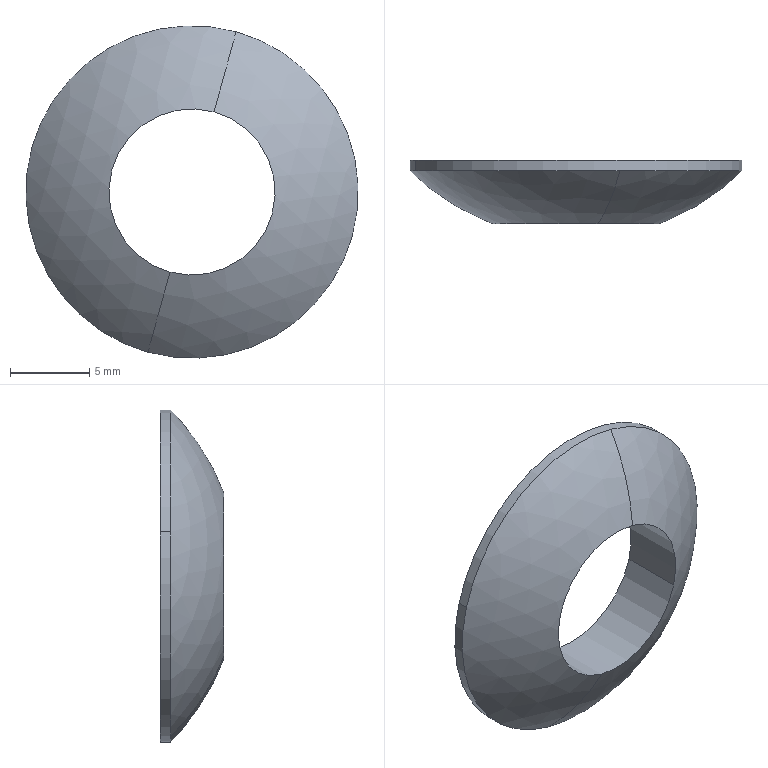Component | SolidWorks | SphericalWasherA21-3 | 1 solid | 7 faces | box 21 x 4 x 21 mm | volume 625 mm3 | cylinder 4 | sphere 2 | plane 1 | commonest cylinder face diameters 21 x2 10.5 x2 | material Nickel
build123d program:
from build123d import *


with BuildPart() as part:
    # Sketch1 → Base-Revolve (revolve)
    with BuildSketch(Plane.XY, mode=Mode.PRIVATE) as base_revolve_sk:
        with BuildLine():
            Line((5.25, 0), (10.5, 0))
            Line((10.5, 0), (10.5, 0.6609))
            ThreePointArc((10.5, 0.6609), (8.05, 2.606), (5.25, 4))
            Line((5.25, 4), (5.25, 0))
        make_face()
    revolve(base_revolve_sk.sketch.rotate(Axis((0, 4.036, 0), (0, -1, 0)), 90), axis=Axis((0, 4.036, 0), (0, -1, 0)))


solid = part.part

# Placed as in the assembly
solid = solid.moved(Location((-96, 234.501, 0), (180, 0, 0)))
STEP:
#1=COLOUR_RGB('',0.7922,0.8196,0.9333);
#2=FILL_AREA_STYLE_COLOUR('',#1);
#3=FILL_AREA_STYLE('',(#2));
#4=SURFACE_STYLE_FILL_AREA(#3);
#5=SURFACE_SIDE_STYLE('',(#4));
#6=SURFACE_STYLE_USAGE(.BOTH.,#5);
#7=PRESENTATION_STYLE_ASSIGNMENT((#6));
#8=CARTESIAN_POINT('',(-4.178,9.232,0.1097));
#9=VERTEX_POINT('',#8);
#10=CARTESIAN_POINT('',(-3.381,9.232,-0.1097));
#11=VERTEX_POINT('',#10);
#12=CARTESIAN_POINT('',(-3.78,9.232,0.));
#13=DIRECTION('',(-0.,-1.,-0.));
#14=DIRECTION('',(-0.9642,0.,0.2653));
#15=AXIS2_PLACEMENT_3D('',#12,#13,#14);
#16=CIRCLE('',#15,0.4134);
#17=EDGE_CURVE('',#9,#11,#16,.T.);
#18=ORIENTED_EDGE('',*,*,#17,.T.);
#19=CARTESIAN_POINT('',(-3.381,9.206,-0.1097));
#20=VERTEX_POINT('',#19);
#21=CARTESIAN_POINT('',(-3.381,9.073,-0.1097));
#22=DIRECTION('',(-0.,-1.,-0.));
#23=VECTOR('',#22,39.37);
#24=LINE('',#21,#23);
#25=EDGE_CURVE('',#11,#20,#24,.T.);
#26=ORIENTED_EDGE('',*,*,#25,.T.);
#27=CARTESIAN_POINT('',(-3.889,9.206,-0.3986));
#28=VERTEX_POINT('',#27);
#29=CARTESIAN_POINT('',(-3.78,9.206,0.));
#30=DIRECTION('',(-0.,-1.,-0.));
#31=DIRECTION('',(-0.9642,0.,0.2653));
#32=AXIS2_PLACEMENT_3D('',#29,#30,#31);
#33=CIRCLE('',#32,0.4134);
#34=EDGE_CURVE('',#28,#20,#33,.T.);
#35=ORIENTED_EDGE('',*,*,#34,.F.);
#36=CARTESIAN_POINT('',(-4.178,9.206,0.1097));
#37=VERTEX_POINT('',#36);
#38=CARTESIAN_POINT('',(-3.78,9.206,0.));
#39=DIRECTION('',(-0.,-1.,-0.));
#40=DIRECTION('',(-0.9642,0.,0.2653));
#41=AXIS2_PLACEMENT_3D('',#38,#39,#40);
#42=CIRCLE('',#41,0.4134);
#43=EDGE_CURVE('',#37,#28,#42,.T.);
#44=ORIENTED_EDGE('',*,*,#43,.F.);
#45=CARTESIAN_POINT('',(-4.178,9.073,0.1097));
#46=DIRECTION('',(-0.,-1.,-0.));
#47=VECTOR('',#46,39.37);
#48=LINE('',#45,#47);
#49=EDGE_CURVE('',#9,#37,#48,.T.);
#50=ORIENTED_EDGE('',*,*,#49,.F.);
#51=EDGE_LOOP('',(#18,#26,#35,#44,#50));
#52=FACE_OUTER_BOUND('',#51,.T.);
#53=CARTESIAN_POINT('',(-3.78,9.073,0.));
#54=DIRECTION('',(-0.,-1.,-0.));
#55=DIRECTION('',(-0.9642,0.,0.2653));
#56=AXIS2_PLACEMENT_3D('',#53,#54,#55);
#57=CYLINDRICAL_SURFACE('',#56,0.4134);
#58=ADVANCED_FACE('',(#52),#57,.T.);
#59=ORIENTED_EDGE('',*,*,#34,.T.);
#60=CARTESIAN_POINT('',(-3.67,9.206,0.3986));
#61=VERTEX_POINT('',#60);
#62=CARTESIAN_POINT('',(-3.78,9.206,0.));
#63=DIRECTION('',(-0.,-1.,-0.));
#64=DIRECTION('',(-0.9642,0.,0.2653));
#65=AXIS2_PLACEMENT_3D('',#62,#63,#64);
#66=CIRCLE('',#65,0.4134);
#67=EDGE_CURVE('',#20,#61,#66,.T.);
#68=ORIENTED_EDGE('',*,*,#67,.T.);
#69=CARTESIAN_POINT('',(-3.725,9.075,0.1993));
#70=VERTEX_POINT('',#69);
#71=CARTESIAN_POINT('',(-3.78,9.628,0.));
#72=DIRECTION('',(0.9642,-0.,-0.2653));
#73=DIRECTION('',(-0.2653,0.,-0.9642));
#74=AXIS2_PLACEMENT_3D('',#71,#72,#73);
#75=CIRCLE('',#74,0.5906);
#76=EDGE_CURVE('',#61,#70,#75,.T.);
#77=ORIENTED_EDGE('',*,*,#76,.T.);
#78=CARTESIAN_POINT('',(-3.58,9.075,-0.05483));
#79=VERTEX_POINT('',#78);
#80=CARTESIAN_POINT('',(-3.78,9.075,0.));
#81=DIRECTION('',(-0.,-1.,-0.));
#82=DIRECTION('',(-0.9642,0.,0.2653));
#83=AXIS2_PLACEMENT_3D('',#80,#81,#82);
#84=CIRCLE('',#83,0.2067);
#85=EDGE_CURVE('',#79,#70,#84,.T.);
#86=ORIENTED_EDGE('',*,*,#85,.F.);
#87=CARTESIAN_POINT('',(-3.834,9.075,-0.1993));
#88=VERTEX_POINT('',#87);
#89=CARTESIAN_POINT('',(-3.78,9.075,0.));
#90=DIRECTION('',(-0.,-1.,-0.));
#91=DIRECTION('',(-0.9642,0.,0.2653));
#92=AXIS2_PLACEMENT_3D('',#89,#90,#91);
#93=CIRCLE('',#92,0.2067);
#94=EDGE_CURVE('',#88,#79,#93,.T.);
#95=ORIENTED_EDGE('',*,*,#94,.F.);
#96=CARTESIAN_POINT('',(-3.78,9.628,0.));
#97=DIRECTION('',(-0.9642,0.,0.2653));
#98=DIRECTION('',(0.2653,0.,0.9642));
#99=AXIS2_PLACEMENT_3D('',#96,#97,#98);
#100=CIRCLE('',#99,0.5906);
#101=EDGE_CURVE('',#28,#88,#100,.T.);
#102=ORIENTED_EDGE('',*,*,#101,.F.);
#103=EDGE_LOOP('',(#59,#68,#77,#86,#95,#102));
#104=FACE_OUTER_BOUND('',#103,.T.);
#105=CARTESIAN_POINT('',(-3.78,9.628,0.));
#106=DIRECTION('',(0.9642,-0.,-0.2653));
#107=DIRECTION('',(-0.2653,0.,-0.9642));
#108=AXIS2_PLACEMENT_3D('',#105,#106,#107);
#109=SPHERICAL_SURFACE('',#108,0.5906);
#110=ADVANCED_FACE('',(#104),#109,.T.);
#111=CARTESIAN_POINT('',(-3.58,9.232,-0.05483));
#112=VERTEX_POINT('',#111);
#113=CARTESIAN_POINT('',(-3.979,9.232,0.05483));
#114=VERTEX_POINT('',#113);
#115=CARTESIAN_POINT('',(-3.78,9.232,0.));
#116=DIRECTION('',(-0.,-1.,-0.));
#117=DIRECTION('',(-0.9642,0.,0.2653));
#118=AXIS2_PLACEMENT_3D('',#115,#116,#117);
#119=CIRCLE('',#118,0.2067);
#120=EDGE_CURVE('',#112,#114,#119,.T.);
#121=ORIENTED_EDGE('',*,*,#120,.F.);
#122=CARTESIAN_POINT('',(-3.58,9.073,-0.05483));
#123=DIRECTION('',(-0.,-1.,-0.));
#124=VECTOR('',#123,39.37);
#125=LINE('',#122,#124);
#126=EDGE_CURVE('',#112,#79,#125,.T.);
#127=ORIENTED_EDGE('',*,*,#126,.T.);
#128=ORIENTED_EDGE('',*,*,#85,.T.);
#129=CARTESIAN_POINT('',(-3.979,9.075,0.05483));
#130=VERTEX_POINT('',#129);
#131=CARTESIAN_POINT('',(-3.78,9.075,0.));
#132=DIRECTION('',(-0.,-1.,-0.));
#133=DIRECTION('',(-0.9642,0.,0.2653));
#134=AXIS2_PLACEMENT_3D('',#131,#132,#133);
#135=CIRCLE('',#134,0.2067);
#136=EDGE_CURVE('',#70,#130,#135,.T.);
#137=ORIENTED_EDGE('',*,*,#136,.T.);
#138=CARTESIAN_POINT('',(-3.979,9.073,0.05483));
#139=DIRECTION('',(-0.,-1.,-0.));
#140=VECTOR('',#139,39.37);
#141=LINE('',#138,#140);
#142=EDGE_CURVE('',#114,#130,#141,.T.);
#143=ORIENTED_EDGE('',*,*,#142,.F.);
#144=EDGE_LOOP('',(#121,#127,#128,#137,#143));
#145=FACE_OUTER_BOUND('',#144,.T.);
#146=CARTESIAN_POINT('',(-3.78,9.073,0.));
#147=DIRECTION('',(-0.,-1.,-0.));
#148=DIRECTION('',(-0.9642,0.,0.2653));
#149=AXIS2_PLACEMENT_3D('',#146,#147,#148);
#150=CYLINDRICAL_SURFACE('',#149,0.2067);
#151=ADVANCED_FACE('',(#145),#150,.F.);
#152=ORIENTED_EDGE('',*,*,#126,.F.);
#153=CARTESIAN_POINT('',(-3.78,9.232,0.));
#154=DIRECTION('',(-0.,-1.,-0.));
#155=DIRECTION('',(-0.9642,0.,0.2653));
#156=AXIS2_PLACEMENT_3D('',#153,#154,#155);
#157=CIRCLE('',#156,0.2067);
#158=EDGE_CURVE('',#114,#112,#157,.T.);
#159=ORIENTED_EDGE('',*,*,#158,.F.);
#160=ORIENTED_EDGE('',*,*,#142,.T.);
#161=CARTESIAN_POINT('',(-3.78,9.075,0.));
#162=DIRECTION('',(-0.,-1.,-0.));
#163=DIRECTION('',(-0.9642,0.,0.2653));
#164=AXIS2_PLACEMENT_3D('',#161,#162,#163);
#165=CIRCLE('',#164,0.2067);
#166=EDGE_CURVE('',#130,#88,#165,.T.);
#167=ORIENTED_EDGE('',*,*,#166,.T.);
#168=ORIENTED_EDGE('',*,*,#94,.T.);
#169=EDGE_LOOP('',(#152,#159,#160,#167,#168));
#170=FACE_OUTER_BOUND('',#169,.T.);
#171=CARTESIAN_POINT('',(-3.78,9.073,0.));
#172=DIRECTION('',(-0.,-1.,-0.));
#173=DIRECTION('',(-0.9642,0.,0.2653));
#174=AXIS2_PLACEMENT_3D('',#171,#172,#173);
#175=CYLINDRICAL_SURFACE('',#174,0.2067);
#176=ADVANCED_FACE('',(#170),#175,.F.);
#177=ORIENTED_EDGE('',*,*,#76,.F.);
#178=CARTESIAN_POINT('',(-3.78,9.206,0.));
#179=DIRECTION('',(-0.,-1.,-0.));
#180=DIRECTION('',(-0.9642,0.,0.2653));
#181=AXIS2_PLACEMENT_3D('',#178,#179,#180);
#182=CIRCLE('',#181,0.4134);
#183=EDGE_CURVE('',#61,#37,#182,.T.);
#184=ORIENTED_EDGE('',*,*,#183,.T.);
#185=ORIENTED_EDGE('',*,*,#43,.T.);
#186=ORIENTED_EDGE('',*,*,#101,.T.);
#187=ORIENTED_EDGE('',*,*,#166,.F.);
#188=ORIENTED_EDGE('',*,*,#136,.F.);
#189=EDGE_LOOP('',(#177,#184,#185,#186,#187,#188));
#190=FACE_OUTER_BOUND('',#189,.T.);
#191=CARTESIAN_POINT('',(-3.78,9.628,0.));
#192=DIRECTION('',(0.9642,-0.,-0.2653));
#193=DIRECTION('',(-0.2653,0.,-0.9642));
#194=AXIS2_PLACEMENT_3D('',#191,#192,#193);
#195=SPHERICAL_SURFACE('',#194,0.5906);
#196=ADVANCED_FACE('',(#190),#195,.T.);
#197=ORIENTED_EDGE('',*,*,#25,.F.);
#198=CARTESIAN_POINT('',(-3.78,9.232,0.));
#199=DIRECTION('',(-0.,-1.,-0.));
#200=DIRECTION('',(-0.9642,0.,0.2653));
#201=AXIS2_PLACEMENT_3D('',#198,#199,#200);
#202=CIRCLE('',#201,0.4134);
#203=EDGE_CURVE('',#11,#9,#202,.T.);
#204=ORIENTED_EDGE('',*,*,#203,.T.);
#205=ORIENTED_EDGE('',*,*,#49,.T.);
#206=ORIENTED_EDGE('',*,*,#183,.F.);
#207=ORIENTED_EDGE('',*,*,#67,.F.);
#208=EDGE_LOOP('',(#197,#204,#205,#206,#207));
#209=FACE_OUTER_BOUND('',#208,.T.);
#210=CARTESIAN_POINT('',(-3.78,9.073,0.));
#211=DIRECTION('',(-0.,-1.,-0.));
#212=DIRECTION('',(-0.9642,0.,0.2653));
#213=AXIS2_PLACEMENT_3D('',#210,#211,#212);
#214=CYLINDRICAL_SURFACE('',#213,0.4134);
#215=ADVANCED_FACE('',(#209),#214,.T.);
#216=ORIENTED_EDGE('',*,*,#17,.F.);
#217=ORIENTED_EDGE('',*,*,#203,.F.);
#218=EDGE_LOOP('',(#216,#217));
#219=FACE_OUTER_BOUND('',#218,.T.);
#220=ORIENTED_EDGE('',*,*,#158,.T.);
#221=ORIENTED_EDGE('',*,*,#120,.T.);
#222=EDGE_LOOP('',(#220,#221));
#223=FACE_BOUND('',#222,.T.);
#224=CARTESIAN_POINT('',(-3.834,9.232,-0.1993));
#225=DIRECTION('',(-0.,-1.,-0.));
#226=DIRECTION('',(-0.9642,0.,0.2653));
#227=AXIS2_PLACEMENT_3D('',#224,#225,#226);
#228=PLANE('',#227);
#229=ADVANCED_FACE('',(#219,#223),#228,.F.);
#230=CLOSED_SHELL('',(#58,#110,#151,#176,#196,#215,#229));
#231=MANIFOLD_SOLID_BREP('',#230);
#232=STYLED_ITEM('',(#7),#231);
#233=PRESENTATION_LAYER_ASSIGNMENT('','',(#232));
#234=CARTESIAN_POINT('',(0.,0.,0.));
#235=DIRECTION('',(0.,0.,1.));
#236=DIRECTION('',(1.,0.,0.));
#237=AXIS2_PLACEMENT_3D('',#234,#235,#236);
#238=(LENGTH_UNIT()NAMED_UNIT(*)SI_UNIT($,.METRE.));
#239=LENGTH_MEASURE_WITH_UNIT(LENGTH_MEASURE(0.0254),#238);
#240=DIMENSIONAL_EXPONENTS(1.,0.,0.,0.,0.,0.,0.);
#241=(CONVERSION_BASED_UNIT('',#239)LENGTH_UNIT()NAMED_UNIT(#240));
#242=UNCERTAINTY_MEASURE_WITH_UNIT(LENGTH_MEASURE(0.00001),#241,'','');
#243=(NAMED_UNIT(*)PLANE_ANGLE_UNIT()SI_UNIT($,.RADIAN.));
#244=(NAMED_UNIT(*)SI_UNIT($,.STERADIAN.)SOLID_ANGLE_UNIT());
#245=(GEOMETRIC_REPRESENTATION_CONTEXT(3)GLOBAL_UNCERTAINTY_ASSIGNED_CONTEXT((#242))GLOBAL_UNIT_ASSIGNED_CONTEXT((#241,#243,#244))REPRESENTATION_CONTEXT('',''));
#246=ADVANCED_BREP_SHAPE_REPRESENTATION('',(#231,#237),#245);
#247=(LENGTH_UNIT()NAMED_UNIT(*)SI_UNIT($,.METRE.));
#248=LENGTH_MEASURE_WITH_UNIT(LENGTH_MEASURE(0.0254),#247);
#249=DIMENSIONAL_EXPONENTS(1.,0.,0.,0.,0.,0.,0.);
#250=(CONVERSION_BASED_UNIT('',#248)LENGTH_UNIT()NAMED_UNIT(#249));
#251=UNCERTAINTY_MEASURE_WITH_UNIT(LENGTH_MEASURE(0.00001),#250,'','');
#252=(NAMED_UNIT(*)PLANE_ANGLE_UNIT()SI_UNIT($,.RADIAN.));
#253=(NAMED_UNIT(*)SI_UNIT($,.STERADIAN.)SOLID_ANGLE_UNIT());
#254=(GEOMETRIC_REPRESENTATION_CONTEXT(3)GLOBAL_UNCERTAINTY_ASSIGNED_CONTEXT((#251))GLOBAL_UNIT_ASSIGNED_CONTEXT((#250,#252,#253))REPRESENTATION_CONTEXT('',''));
#255=MECHANICAL_DESIGN_GEOMETRIC_PRESENTATION_REPRESENTATION('',(#232),#254);